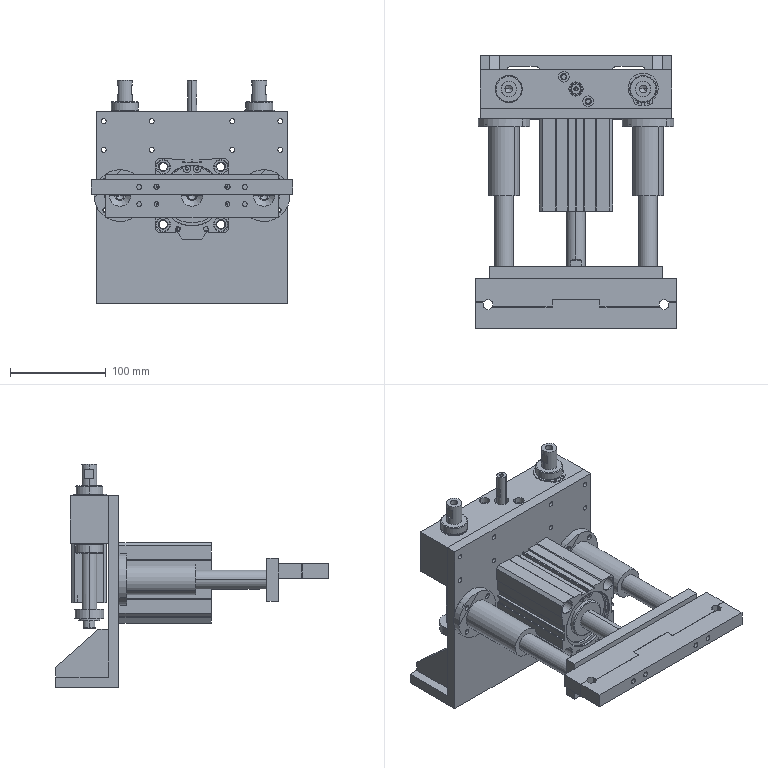Assembly | SolidWorks | mm | 28 component files | 28 solids | 1169 faces | box 210 x 284.11 x 232.5 mm | volume 1844590 mm3 | cylinder 548 | plane 431 | cone 160 | torus 18 | spline 12 | commonest cylinder face diameters 0.4 x45 5 x38 11 x38 0.8 x29 6.6 x28 2 x26 5.5 x24 20 x21
Bill of materials:
16mmLinearBearingSnapRingTypeLmuwm16_2_03 | 2 |  | Thick-walled cylindrical tube or sleeve with a plain through-bore and two shallow circumferential grooves, one near each end.
28mmShaftSnapRingGB896-1986-28 | 2 |  | Thin, flat, open (split) ring with two widened lugs on either side of the gap, each lug having a small round hole. The shape resembles an external retaining ring.
8mmLargeWasher | 2 |  | Flat circular disc with a concentric round through-hole, like a plain washer.
ACQS_20x60_60r | 1 |  | Long slender cylindrical shaft with a small axial hole and flats at one end, on top of a larger cylindrical collar and a short stepped base carrying several circumferential grooves or flanges.
ACQS_20x6060_b | 1 |  | Tall prismatic body with a nearly square cross-section and chamfered corners. It has two diagonal-corner through-holes, a central circular bore with counterbore or ring recesses, and dovetail- or T-shaped slots running along its length on one corner region.
ACQS_63x50_50r | 1 |  | Disc-shaped head with several circumferential grooves on its rim and a cylindrical rod projecting from one face. The rod end has a small axial hole and a flat.
ACQS_63x5050_b | 1 |  | Block-shaped prismatic body with a square end profile, four corner through-holes with counterbore rings, a large central circular recess with a concentric boss, and several longitudinal slots and grooves along its sides.
CS1_G | 2 |  | Elongated rectangular bar with rounded edges, a cylindrical stub projecting from one end, a narrow rail or tongue along its underside, and a small round boss or screw head near the opposite end on the underside.
LinearBearing20mmStandardRoundFlangeDoubleLinerTypeLMF20LUU | 2 |  | Hollow cylindrical tube with a circular flange at one end. The flange has four small through-holes on a square pattern.
M8x14HexSocket | 2 |  | Stepped cylindrical pin: a short larger-diameter base with a rounded bottom edge and a smaller-diameter cylindrical shank with a chamfered top end.
YS01-053FixedBracket2 | 1 |  | L-shaped bracket: a large flat vertical plate with many round holes, joined to a short horizontal foot with a chamfered or angled profile. The foot has four elongated slots.
YS01-054ClampingBlockMountingPlate | 1 |  | Flat rectangular bar or plate with three countersunk or counterbored through-holes along its centerline and two groups of four small through-holes between them.
YS01-055GuideRod2 | 2 |  | Straight, plain cylindrical tube: a long round body with a central axial bore and flat square-cut ends.
YS01-056LiftingBearingHousing-ClampingAssembly | 1 |  | Rectangular bar-shaped block with a rectangular notch cut into the center of one long edge (bridge/U-like profile), two large through holes near the ends, a central group of three smaller holes, and a pattern of small holes on the large side face.
YS01-057LiftingGuideRod | 2 |  | Slender cylindrical tube with an axial bore and a pair of shallow opposite flats (or a shallow pocket) near one end.
YS01-058BufferPad | 2 |  | Thick plain annular ring (spacer/washer-like shape) with a concentric through hole and flat parallel faces.
YS01-059CylinderExtensionRod | 1 |  | Stepped cylindrical shaft/tube: a larger-diameter main body with an axial bore at one end, a smaller-diameter coaxial spigot at the other end, and a pair of shallow opposite flats on the main body.
YS01-071NozzleFasteningClampBlock | 1 |  | Long rectangular bar with a profiled edge: two raised pads separated by a central recess, small V/chamfered notches near each end, and four countersunk holes through the side face arranged in two pairs.
YS01-072NozzleFasteningClampBlock2 | 1 |  | Long rectangular bar with a profiled edge: a central raised boss on one long edge, V-shaped notches near each end, and four plain through holes on the side face in two pairs.
Mates:
1. coincident | LinearBearing20mmStandardRoundFlangeDoubleLinerTypeLMF20LUU-1 face at (-641.612, -154.873, 2398.4) dir (0, 1, 0) | YS01-053FixedBracket2-1 face at (-566.612, -154.873, 2398.4) dir (0, -1, 0)
2. coincident | YS01-053FixedBracket2-1 face at (-566.612, -154.873, 2398.4) dir (0, -1, 0) | LinearBearing20mmStandardRoundFlangeDoubleLinerTypeLMF20LUU-2 face at (-491.612, -154.873, 2398.4) dir (0, 1, 0)
3. angle | YS01-053FixedBracket2-1 face at (-666.612, -143.873, 2285.9) dir (-1, 0, 0) | LinearBearing20mmStandardRoundFlangeDoubleLinerTypeLMF20LUU-1 face at (-674.504, -162.863, 2390.964) dir (-0.7071, 0, 0.7071)
4. concentric | YS01-053FixedBracket2-1 face at (-506.815, -154.873, 2413.603) dir (0, -1, 0) r 2.1 | LinearBearing20mmStandardRoundFlangeDoubleLinerTypeLMF20LUU-2 face at (-506.815, -154.873, 2413.603) dir (0, 1, 0) r 2.75
5. concentric | YS01-055GuideRod2-1 face at (-641.612, -143.873, 2398.4) dir (0, -1, 0) r 10 | LinearBearing20mmStandardRoundFlangeDoubleLinerTypeLMF20LUU-1 face at (-641.612, -234.873, 2398.4) dir (0, 1, 0) r 16
6. concentric | YS01-055GuideRod2-2 face at (-491.612, -143.873, 2398.4) dir (0, -1, 0) r 10 | LinearBearing20mmStandardRoundFlangeDoubleLinerTypeLMF20LUU-2 face at (-491.612, -234.873, 2398.4) dir (0, 1, 0) r 16
7. coincident | YS01-055GuideRod2-2 face at (-491.612, -308.873, 2398.4) dir (0, -1, 0) | YS01-054ClampingBlockMountingPlate-2 face at (-589.112, -308.873, 2343.9) dir (0, 1, 0)
8. concentric | YS01-055GuideRod2-2 face at (-491.612, -308.873, 2398.4) dir (0, -1, 0) r 4.25 | YS01-054ClampingBlockMountingPlate-2 face at (-491.612, -320.873, 2398.4) dir (0, -1, 0) r 5.5
9. coincident | ACQS_63x50_G_2_50-1/ACQS_63x50_50r-1 face at (-566.612, -308.873, 2398.4) dir (0, -1, 0) | YS01-054ClampingBlockMountingPlate-2 face at (-589.112, -308.873, 2343.9) dir (0, 1, 0)
10. concentric | ACQS_63x50_G_2_50-1/ACQS_63x50_50r-1 face at (-566.612, -300.873, 2398.4) dir (0, -1, 0) r 10 | YS01-054ClampingBlockMountingPlate-2 face at (-566.612, -320.873, 2398.4) dir (0, -1, 0) r 5.5
11. concentric | YS01-056LiftingBearingHousing-ClampingAssembly-1 face at (-636.612, -123.873, 2436.1) dir (0, 0, 1) r 14 | 16mmLinearBearingSnapRingTypeLmuwm16_2_03-1 face at (-636.612, -123.873, 2461) dir (0, 0, -1) r 14
12. coincident | YS01-056LiftingBearingHousing-ClampingAssembly-1 face at (-466.612, -103.873, 2436.1) dir (0, 0, -1) | 16mmLinearBearingSnapRingTypeLmuwm16_2_03-1 face at (-636.612, -110.123, 2436.1) dir (0, 0, -1)
13. concentric | YS01-056LiftingBearingHousing-ClampingAssembly-1 face at (-496.612, -123.873, 2436.1) dir (0, 0, 1) r 14 | 16mmLinearBearingSnapRingTypeLmuwm16_2_03-2 face at (-496.612, -123.873, 2461) dir (0, 0, -1) r 14
14. coincident | YS01-056LiftingBearingHousing-ClampingAssembly-1 face at (-466.612, -103.873, 2485.9) dir (0, 0, 1) | 16mmLinearBearingSnapRingTypeLmuwm16_2_03-2 face at (-496.612, -110.123, 2485.9) dir (0, 0, 1)
15. coincident | YS01-053FixedBracket2-1 face at (-666.612, -143.873, 2485.9) dir (0, 0, 1) | YS01-056LiftingBearingHousing-ClampingAssembly-1 face at (-466.612, -103.873, 2485.9) dir (0, 0, 1)
16. coincident | YS01-053FixedBracket2-1 face at (-566.612, -143.873, 2398.4) dir (0, 1, 0) | YS01-056LiftingBearingHousing-ClampingAssembly-1 face at (-566.612, -143.873, 2388.4) dir (0, -1, 0)
17. concentric | YS01-056LiftingBearingHousing-ClampingAssembly-1 face at (-566.612, -123.873, 2436.1) dir (0, 0, 1) r 7.5 | ACQS_20x60_0-2/ACQS_20x60_60r-1 face at (-566.612, -123.873, 2465.9) dir (0, 0, 1) r 5
18. coincident | YS01-056LiftingBearingHousing-ClampingAssembly-1 face at (-546.612, -143.873, 2465.9) dir (0, 0, -1) | ACQS_20x60_0-2/ACQS_20x6060_b-1 face at (-559.063, -106.646, 2465.9) dir (0, 0, 1)
19. concentric | YS01-059CylinderExtensionRod-2 face at (-566.612, -123.873, 2518.4) dir (0, 0, -1) r 5 | ACQS_20x60_0-2/ACQS_20x60_60r-1 face at (-566.612, -123.873, 2465.9) dir (0, 0, 1) r 5
20. coincident | YS01-059CylinderExtensionRod-2 face at (-566.612, -123.873, 2470.4) dir (0, 0, -1) | ACQS_20x60_0-2/ACQS_20x60_60r-1 face at (-566.612, -123.873, 2470.4) dir (0, 0, 1)
21. concentric | 8mmLargeWasher-1 face at (-496.612, -123.873, 2355.4) dir (0, 0, 1) r 4.25 | M8x14HexSocket-1 face at (-496.612, -123.873, 2369.4) dir (0, 0, -1) r 4
22. coincident | 8mmLargeWasher-1 face at (-496.612, -123.873, 2355.4) dir (0, 0, -1) | M8x14HexSocket-1 face at (-496.612, -123.873, 2355.4) dir (0, 0, 1)
23. concentric | YS01-058BufferPad-2 face at (-636.612, -123.873, 2367.4) dir (0, 0, -1) r 15 | 8mmLargeWasher-2 face at (-636.612, -123.873, 2355.4) dir (0, 0, 1) r 4.25
24. coincident | YS01-058BufferPad-2 face at (-636.612, -123.873, 2357.4) dir (0, 0, -1) | 8mmLargeWasher-2 face at (-636.612, -123.873, 2357.4) dir (0, 0, 1)
25. concentric | M8x14HexSocket-2 face at (-636.612, -123.873, 2369.4) dir (0, 0, -1) r 4 | 8mmLargeWasher-2 face at (-636.612, -123.873, 2355.4) dir (0, 0, 1) r 4.25
26. coincident | M8x14HexSocket-2 face at (-636.612, -123.873, 2355.4) dir (0, 0, 1) | 8mmLargeWasher-2 face at (-636.612, -123.873, 2355.4) dir (0, 0, -1)
27. concentric | 16mmLinearBearingSnapRingTypeLmuwm16_2_03-2 face at (-496.612, -123.873, 2486.7) dir (0, 0, -1) r 13.5 | 28mmShaftSnapRingGB896-1986-28-1 face at (-496.612, -123.873, 2485.9) dir (0, 0, 1) r 13.5
28. coincident | 16mmLinearBearingSnapRingTypeLmuwm16_2_03-2 face at (-496.612, -110.123, 2485.9) dir (0, 0, 1) | 28mmShaftSnapRingGB896-1986-28-1 face at (-496.612, -123.873, 2485.9) dir (0, 0, -1)
29. coincident | 16mmLinearBearingSnapRingTypeLmuwm16_2_03-2 face at (-496.612, -110.123, 2434.5) dir (0, 0, 1) | 28mmShaftSnapRingGB896-1986-28-2 face at (-496.612, -123.873, 2434.5) dir (0, 0, -1)
30. concentric | 16mmLinearBearingSnapRingTypeLmuwm16_2_03-2 face at (-496.612, -123.873, 2435.3) dir (0, 0, -1) r 13.5 | 28mmShaftSnapRingGB896-1986-28-2 face at (-496.612, -123.873, 2434.5) dir (0, 0, 1) r 13.5
31. coincident | 8mmLargeWasher-1 face at (-496.612, -123.873, 2357.4) dir (0, 0, 1) | YS01-057LiftingGuideRod-1 face at (-496.612, -123.873, 2357.4) dir (0, 0, -1)
32. concentric | 16mmLinearBearingSnapRingTypeLmuwm16_2_03-1 face at (-636.612, -123.873, 2461) dir (0, 0, -1) r 8 | YS01-057LiftingGuideRod-2 face at (-636.612, -123.873, 2518.4) dir (0, 0, -1) r 8
33. coincident | YS01-057LiftingGuideRod-1 face at (-496.612, -123.873, 2518.4) dir (0, 0, 1) | YS01-057LiftingGuideRod-2 face at (-636.612, -123.873, 2518.4) dir (0, 0, 1)
34. coincident | ACQS_20x6060_b-1 axis at (-80.9, 0, 0) dir (1, 0, 0) | ACQS_20x60_60r-1 axis at (80.9, 0, 0) dir (-1, 0, 0)
35. coincident | ACQS_20x6060_b-1 axis at (-80.9, 0, 0) dir (1, 0, 0) | ACQS_20x60_60r-1 axis at (80.9, 0, 0) dir (-1, 0, 0)
36. angle | ACQS_20x60_60r-1 plane at (0, 0, 0) dir (0, 0, -1) | ACQS_20x6060_b-1 plane at (0, 0, 0) dir (0, 1, 0)
37. coincident | ACQS_63x5050_b-1 axis at (-80.9, 0, 0) dir (1, 0, 0) | ACQS_63x50_50r-1 axis at (30.9, 0, 0) dir (-1, 0, 0)
38. coincident | ACQS_63x5050_b-1 axis at (-80.9, 0, 0) dir (1, 0, 0) | ACQS_63x50_50r-1 axis at (30.9, 0, 0) dir (-1, 0, 0)
39. angle | ACQS_63x50_50r-1 plane at (-50, 0, 0) dir (0, 0, -1) | ACQS_63x5050_b-1 plane at (0, 0, 0) dir (0, 1, 0)